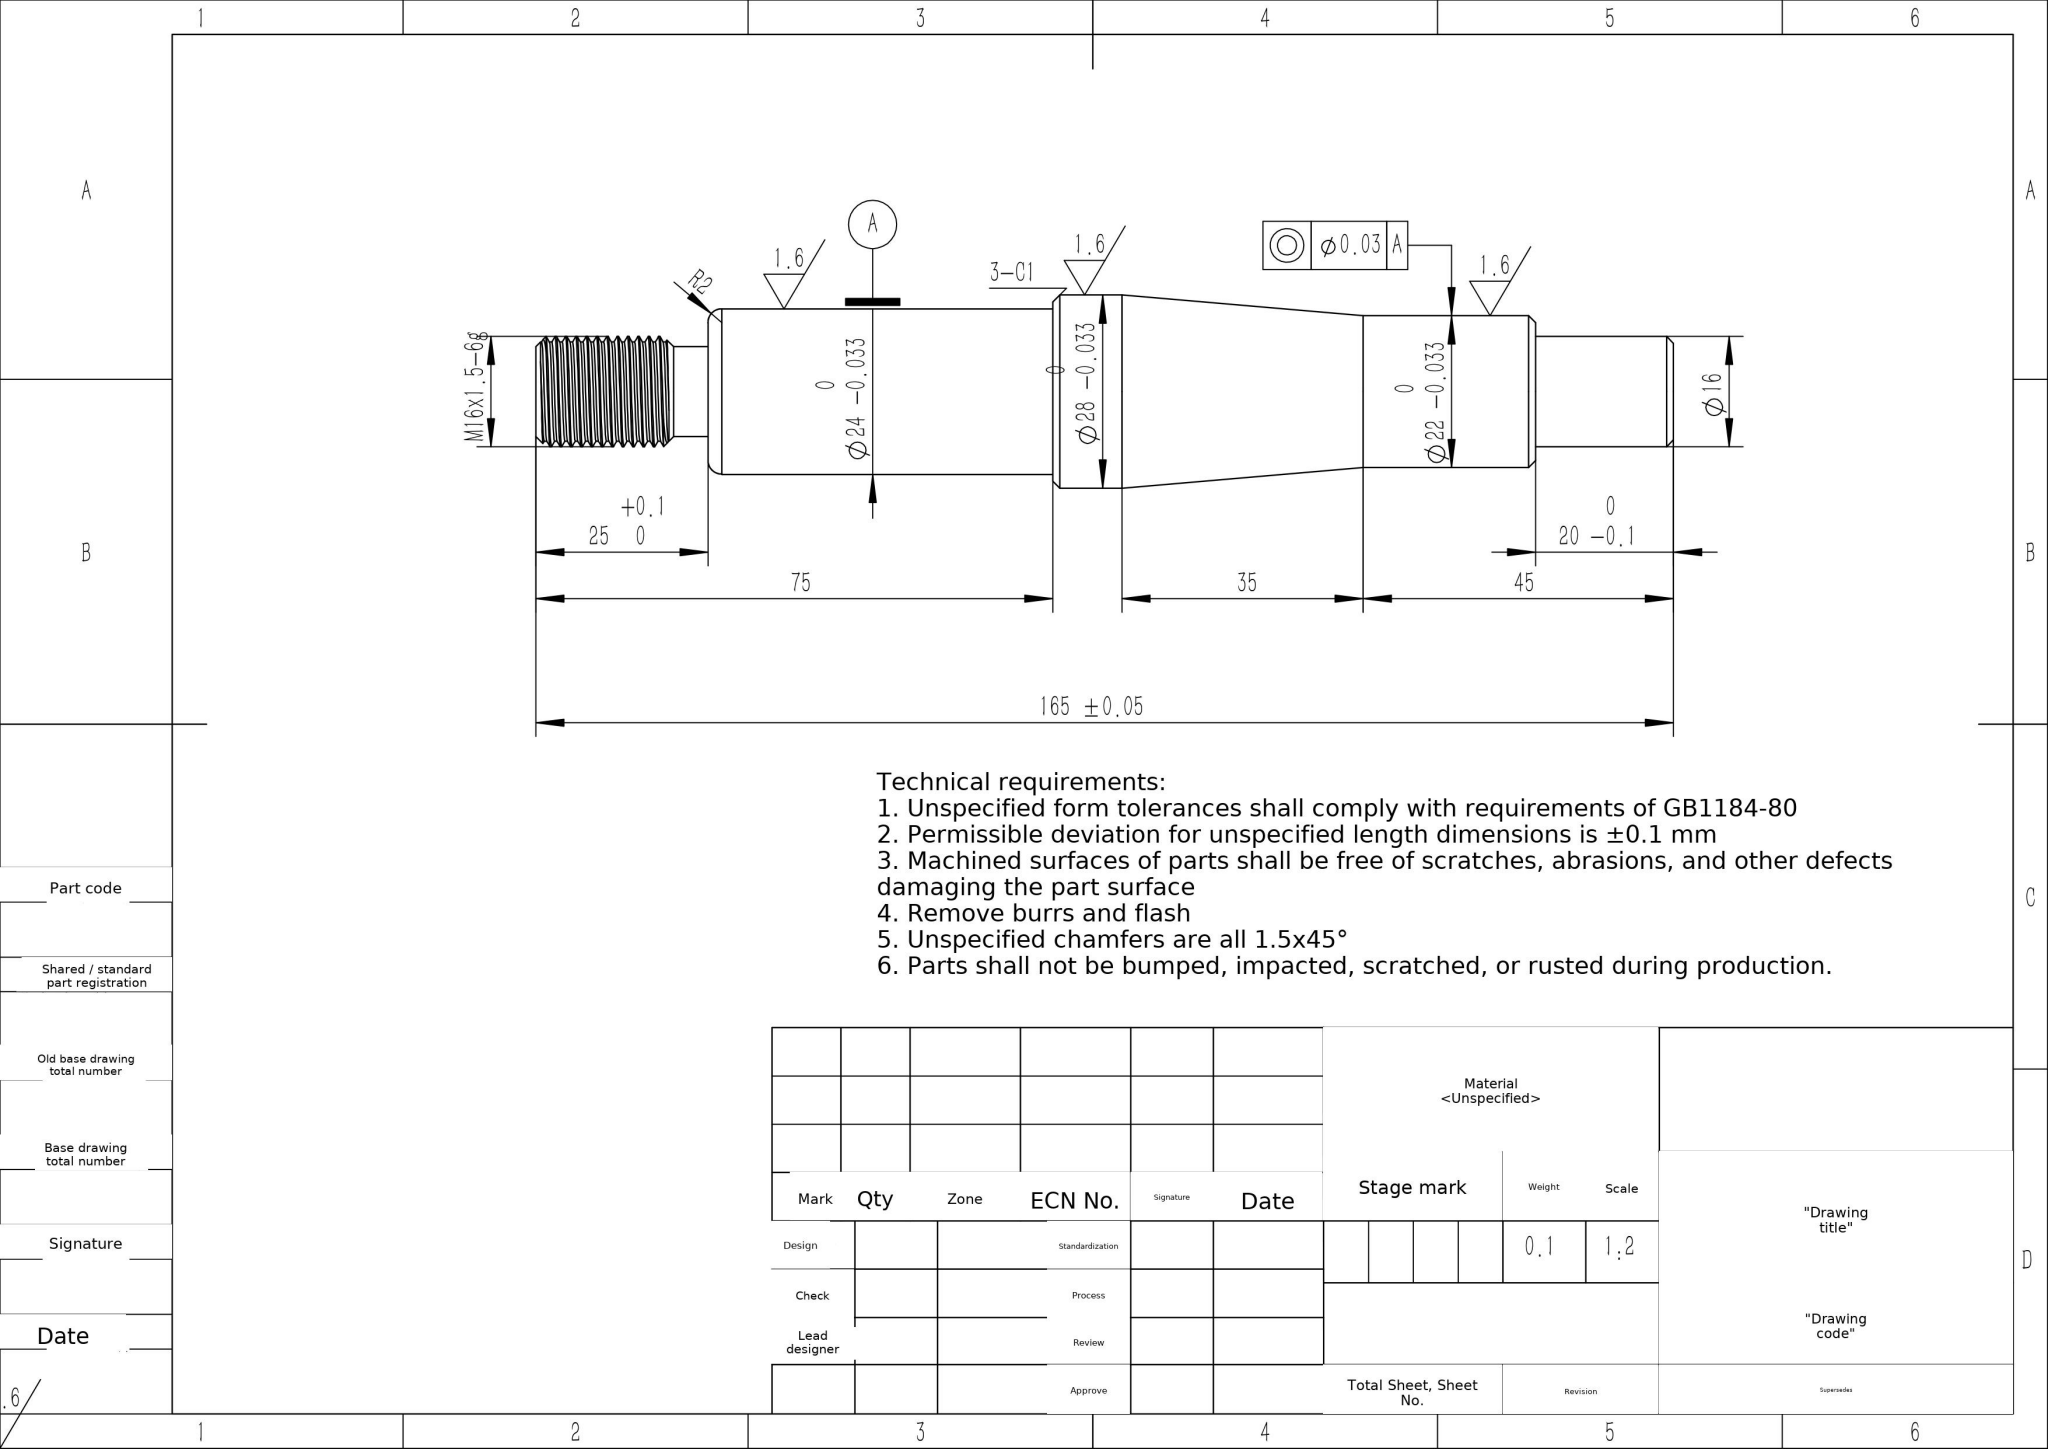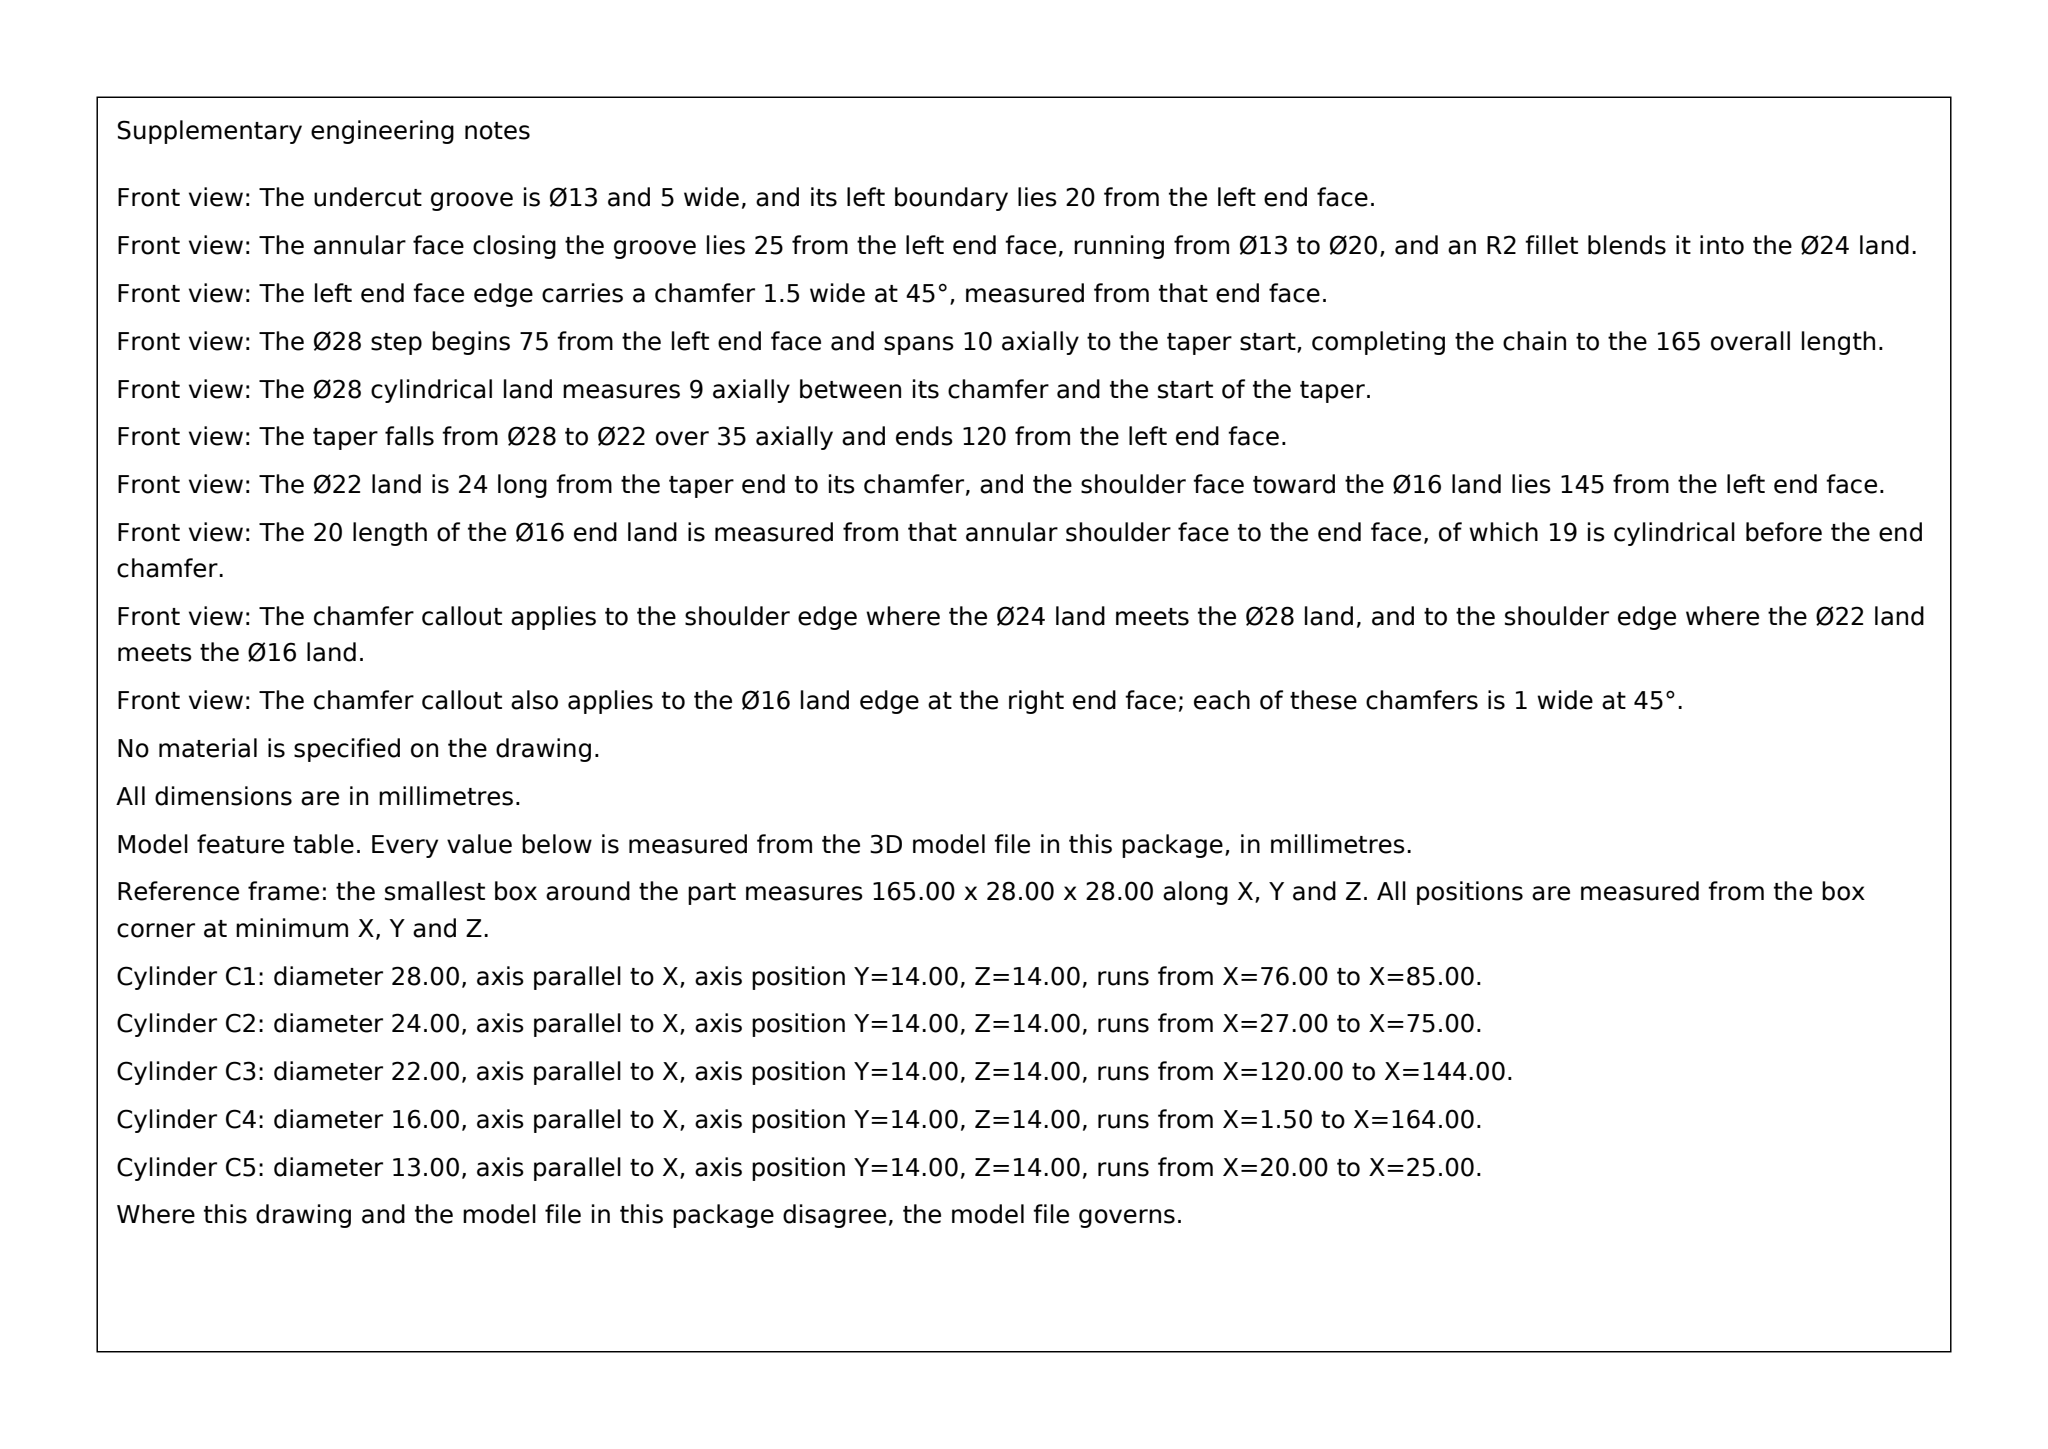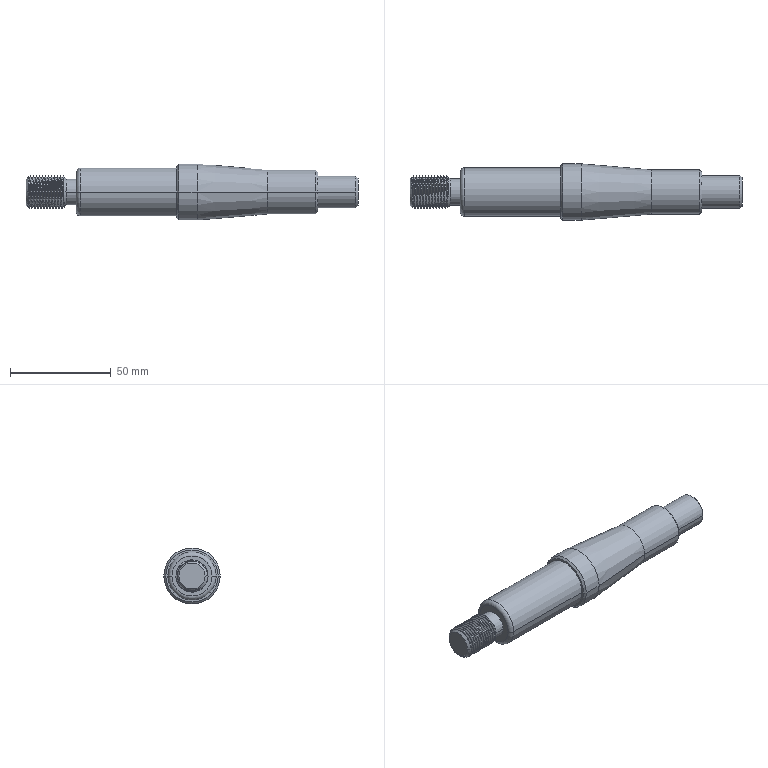Part | SolidWorks | mm | 1 solid | 56 faces | box 165 x 28 x 28 mm | volume 63603 mm3 | cylinder 34 | cone 12 | plane 5 | spline 3 | torus 2 | commonest cylinder face diameters 16 x26 22 x2 28 x2 24 x2 13 x2
Drawing notes:
THREAD UNDERCUT 5 WIDE, FROM 20 TO 25 FROM THD END, R2 AT SHLDR | from the solid: Ø13 cyl, axis x, from 20.0 to 25.0 (5 wide); torus minor r=2.0 major r=10.0 at Ø24 shoulder
THREAD UNDERCUT DIA Ø13 (M16x1.5 RELIEF), 1.5 DEEP PER SIDE | from the solid: Ø13 boss/shaft cyl vs M16 major Ø16: (16-13)/2 = 1.5 depth